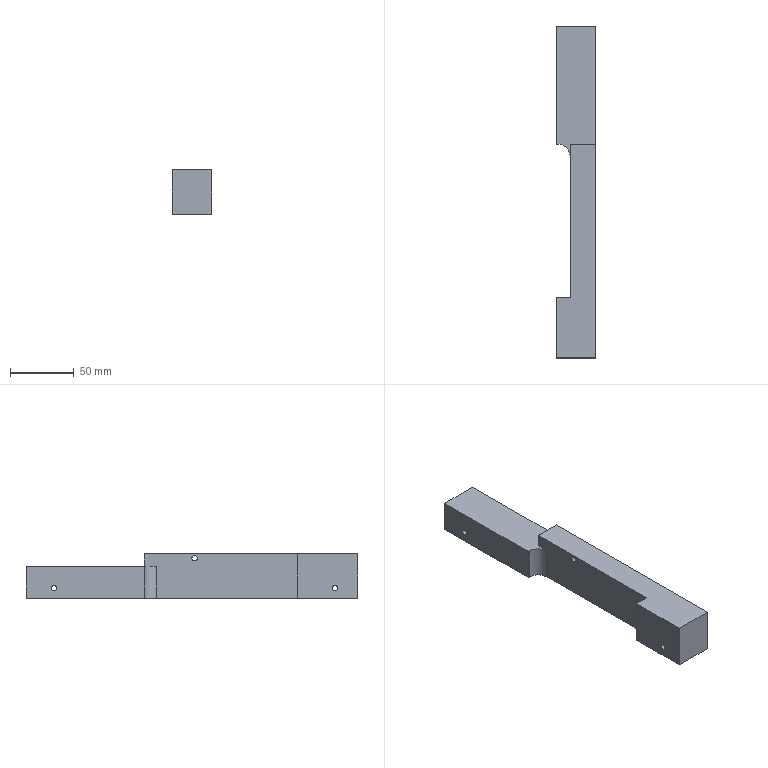Component | SolidWorks | FunnelRotaryCylinderFixingPost-2 | 1 solid | 19 faces | box 31 x 260 x 35 mm | volume 206625 mm3 | plane 12 | cylinder 7 | commonest cylinder face diameters 4.2 x6 20 x1
build123d program:
from build123d import *

# Parameters (mm, degrees)
SKETCH2_W           = 31
SKETCH2_H           = 260
BOSS_EXTRUDE1_DEPTH = 25
SKETCH3_W           = 31
SKETCH3_H           = 167.5
BOSS_EXTRUDE2_DEPTH = 10
M5_TAPPED_HOLE1_D   = 4.2
SKETCH7_W           = 11
SKETCH7_H           = 120
CUT_EXTRUDE1_DEPTH  = 40
FILLET1_R           = 10


with BuildPart() as part:
    # Sketch2 → Boss-Extrude1 (new body)
    with BuildSketch(Plane.XY):
        with Locations((0.5, -69.763)):
            Rectangle(SKETCH2_W, SKETCH2_H)
    extrude(amount=BOSS_EXTRUDE1_DEPTH)

    # Sketch3 → Boss-Extrude2 (add)
    with BuildSketch(Plane(origin=(0, 0, 0), x_dir=(-1, 0, 0), z_dir=(0, 0, -1))):
        with Locations((-0.5, -116.013)):
            Rectangle(SKETCH3_W, SKETCH3_H)
    extrude(amount=BOSS_EXTRUDE2_DEPTH)

    # M5 Tapped Hole1 (through all)
    with Locations(Plane.ZY.offset(15)):
        with Locations((17, 38.237), (-6.5, -71.763), (17, -181.763)):
            Hole(M5_TAPPED_HOLE1_D / 2)

    # Sketch7 → Cut-Extrude1 (cut)
    with BuildSketch(Plane(origin=(0, 0, -10), x_dir=(-1, 0, 0), z_dir=(0, 0, -1))):
        with Locations((-10.5, -92.263)):
            Rectangle(SKETCH7_W, SKETCH7_H)
    extrude(amount=-CUT_EXTRUDE1_DEPTH, mode=Mode.SUBTRACT)

    # Fillet1
    fillet1_edges = [part.edges().sort_by_distance(p)[0] for p in [
        (5, -32.263, 12.5),
    ]]
    fillet(fillet1_edges, radius=FILLET1_R)


solid = part.part

# Placed as in the assembly
solid = solid.moved(Location((-550.496, 52.112, 289.126), (-180, 0, 180)))
STEP:
#1=COLOUR_RGB('',0.7922,0.8196,0.9333);
#2=FILL_AREA_STYLE_COLOUR('',#1);
#3=FILL_AREA_STYLE('',(#2));
#4=SURFACE_STYLE_FILL_AREA(#3);
#5=SURFACE_SIDE_STYLE('',(#4));
#6=SURFACE_STYLE_USAGE(.BOTH.,#5);
#7=PRESENTATION_STYLE_ASSIGNMENT((#6));
#8=CARTESIAN_POINT('',(-22.303,3.557,10.796));
#9=VERTEX_POINT('',#8);
#10=CARTESIAN_POINT('',(-22.303,3.557,10.631));
#11=VERTEX_POINT('',#10);
#12=CARTESIAN_POINT('',(-22.303,3.557,10.714));
#13=DIRECTION('',(1.,0.,0.));
#14=DIRECTION('',(0.,0.,-1.));
#15=AXIS2_PLACEMENT_3D('',#12,#13,#14);
#16=CIRCLE('',#15,0.08268);
#17=EDGE_CURVE('',#9,#11,#16,.T.);
#18=ORIENTED_EDGE('',*,*,#17,.F.);
#19=CARTESIAN_POINT('',(-21.083,3.557,10.796));
#20=VERTEX_POINT('',#19);
#21=CARTESIAN_POINT('',(-21.083,3.557,10.796));
#22=DIRECTION('',(1.,0.,0.));
#23=VECTOR('',#22,39.37);
#24=LINE('',#21,#23);
#25=EDGE_CURVE('',#9,#20,#24,.T.);
#26=ORIENTED_EDGE('',*,*,#25,.T.);
#27=CARTESIAN_POINT('',(-21.083,3.557,10.631));
#28=VERTEX_POINT('',#27);
#29=CARTESIAN_POINT('',(-21.083,3.557,10.714));
#30=DIRECTION('',(1.,0.,0.));
#31=DIRECTION('',(0.,0.,-1.));
#32=AXIS2_PLACEMENT_3D('',#29,#30,#31);
#33=CIRCLE('',#32,0.08268);
#34=EDGE_CURVE('',#20,#28,#33,.T.);
#35=ORIENTED_EDGE('',*,*,#34,.T.);
#36=CARTESIAN_POINT('',(-21.083,3.557,10.631));
#37=DIRECTION('',(1.,0.,0.));
#38=VECTOR('',#37,39.37);
#39=LINE('',#36,#38);
#40=EDGE_CURVE('',#11,#28,#39,.T.);
#41=ORIENTED_EDGE('',*,*,#40,.F.);
#42=EDGE_LOOP('',(#18,#26,#35,#41));
#43=FACE_OUTER_BOUND('',#42,.T.);
#44=CARTESIAN_POINT('',(-21.083,3.557,10.714));
#45=DIRECTION('',(1.,0.,0.));
#46=DIRECTION('',(0.,0.,-1.));
#47=AXIS2_PLACEMENT_3D('',#44,#45,#46);
#48=CYLINDRICAL_SURFACE('',#47,0.08268);
#49=ADVANCED_FACE('',(#43),#48,.F.);
#50=CARTESIAN_POINT('',(-21.87,-0.7737,11.556));
#51=VERTEX_POINT('',#50);
#52=CARTESIAN_POINT('',(-21.87,-0.7737,11.721));
#53=VERTEX_POINT('',#52);
#54=CARTESIAN_POINT('',(-21.87,-0.7737,11.639));
#55=DIRECTION('',(-1.,-0.,-0.));
#56=DIRECTION('',(0.,-1.,0.));
#57=AXIS2_PLACEMENT_3D('',#54,#55,#56);
#58=CIRCLE('',#57,0.08268);
#59=EDGE_CURVE('',#51,#53,#58,.T.);
#60=ORIENTED_EDGE('',*,*,#59,.T.);
#61=CARTESIAN_POINT('',(-21.083,-0.7737,11.721));
#62=VERTEX_POINT('',#61);
#63=CARTESIAN_POINT('',(-21.083,-0.7737,11.721));
#64=DIRECTION('',(1.,0.,0.));
#65=VECTOR('',#64,39.37);
#66=LINE('',#63,#65);
#67=EDGE_CURVE('',#53,#62,#66,.T.);
#68=ORIENTED_EDGE('',*,*,#67,.T.);
#69=CARTESIAN_POINT('',(-21.083,-0.7737,11.556));
#70=VERTEX_POINT('',#69);
#71=CARTESIAN_POINT('',(-21.083,-0.7737,11.639));
#72=DIRECTION('',(1.,0.,0.));
#73=DIRECTION('',(0.,0.,-1.));
#74=AXIS2_PLACEMENT_3D('',#71,#72,#73);
#75=CIRCLE('',#74,0.08268);
#76=EDGE_CURVE('',#62,#70,#75,.T.);
#77=ORIENTED_EDGE('',*,*,#76,.T.);
#78=CARTESIAN_POINT('',(-21.083,-0.7737,11.556));
#79=DIRECTION('',(1.,0.,0.));
#80=VECTOR('',#79,39.37);
#81=LINE('',#78,#80);
#82=EDGE_CURVE('',#51,#70,#81,.T.);
#83=ORIENTED_EDGE('',*,*,#82,.F.);
#84=EDGE_LOOP('',(#60,#68,#77,#83));
#85=FACE_OUTER_BOUND('',#84,.T.);
#86=CARTESIAN_POINT('',(-21.083,-0.7737,11.639));
#87=DIRECTION('',(1.,0.,0.));
#88=DIRECTION('',(0.,0.,-1.));
#89=AXIS2_PLACEMENT_3D('',#86,#87,#88);
#90=CYLINDRICAL_SURFACE('',#89,0.08268);
#91=ADVANCED_FACE('',(#85),#90,.F.);
#92=CARTESIAN_POINT('',(-22.303,-5.104,10.796));
#93=VERTEX_POINT('',#92);
#94=CARTESIAN_POINT('',(-22.303,-5.104,10.631));
#95=VERTEX_POINT('',#94);
#96=CARTESIAN_POINT('',(-22.303,-5.104,10.714));
#97=DIRECTION('',(1.,0.,0.));
#98=DIRECTION('',(0.,0.,-1.));
#99=AXIS2_PLACEMENT_3D('',#96,#97,#98);
#100=CIRCLE('',#99,0.08268);
#101=EDGE_CURVE('',#93,#95,#100,.T.);
#102=ORIENTED_EDGE('',*,*,#101,.F.);
#103=CARTESIAN_POINT('',(-21.083,-5.104,10.796));
#104=VERTEX_POINT('',#103);
#105=CARTESIAN_POINT('',(-21.083,-5.104,10.796));
#106=DIRECTION('',(1.,0.,0.));
#107=VECTOR('',#106,39.37);
#108=LINE('',#105,#107);
#109=EDGE_CURVE('',#93,#104,#108,.T.);
#110=ORIENTED_EDGE('',*,*,#109,.T.);
#111=CARTESIAN_POINT('',(-21.083,-5.104,10.631));
#112=VERTEX_POINT('',#111);
#113=CARTESIAN_POINT('',(-21.083,-5.104,10.714));
#114=DIRECTION('',(1.,0.,0.));
#115=DIRECTION('',(0.,0.,-1.));
#116=AXIS2_PLACEMENT_3D('',#113,#114,#115);
#117=CIRCLE('',#116,0.08268);
#118=EDGE_CURVE('',#104,#112,#117,.T.);
#119=ORIENTED_EDGE('',*,*,#118,.T.);
#120=CARTESIAN_POINT('',(-21.083,-5.104,10.631));
#121=DIRECTION('',(1.,0.,0.));
#122=VECTOR('',#121,39.37);
#123=LINE('',#120,#122);
#124=EDGE_CURVE('',#95,#112,#123,.T.);
#125=ORIENTED_EDGE('',*,*,#124,.F.);
#126=EDGE_LOOP('',(#102,#110,#119,#125));
#127=FACE_OUTER_BOUND('',#126,.T.);
#128=CARTESIAN_POINT('',(-21.083,-5.104,10.714));
#129=DIRECTION('',(1.,0.,0.));
#130=DIRECTION('',(0.,0.,-1.));
#131=AXIS2_PLACEMENT_3D('',#128,#129,#130);
#132=CYLINDRICAL_SURFACE('',#131,0.08268);
#133=ADVANCED_FACE('',(#127),#132,.F.);
#134=CARTESIAN_POINT('',(-22.303,3.557,10.714));
#135=DIRECTION('',(1.,0.,0.));
#136=DIRECTION('',(0.,0.,-1.));
#137=AXIS2_PLACEMENT_3D('',#134,#135,#136);
#138=CIRCLE('',#137,0.08268);
#139=EDGE_CURVE('',#11,#9,#138,.T.);
#140=ORIENTED_EDGE('',*,*,#139,.T.);
#141=ORIENTED_EDGE('',*,*,#17,.T.);
#142=EDGE_LOOP('',(#140,#141));
#143=FACE_BOUND('',#142,.T.);
#144=CARTESIAN_POINT('',(-22.303,0.7814,10.399));
#145=VERTEX_POINT('',#144);
#146=CARTESIAN_POINT('',(-22.303,4.423,10.399));
#147=VERTEX_POINT('',#146);
#148=CARTESIAN_POINT('',(-22.303,4.423,10.399));
#149=DIRECTION('',(0.,1.,-0.));
#150=VECTOR('',#149,39.37);
#151=LINE('',#148,#150);
#152=EDGE_CURVE('',#145,#147,#151,.T.);
#153=ORIENTED_EDGE('',*,*,#152,.F.);
#154=CARTESIAN_POINT('',(-22.303,0.7814,11.383));
#155=VERTEX_POINT('',#154);
#156=CARTESIAN_POINT('',(-22.303,0.7814,10.202));
#157=DIRECTION('',(-0.,0.,1.));
#158=VECTOR('',#157,39.37);
#159=LINE('',#156,#158);
#160=EDGE_CURVE('',#145,#155,#159,.T.);
#161=ORIENTED_EDGE('',*,*,#160,.T.);
#162=CARTESIAN_POINT('',(-22.303,4.423,11.383));
#163=VERTEX_POINT('',#162);
#164=CARTESIAN_POINT('',(-22.303,4.423,11.383));
#165=DIRECTION('',(0.,1.,-0.));
#166=VECTOR('',#165,39.37);
#167=LINE('',#164,#166);
#168=EDGE_CURVE('',#155,#163,#167,.T.);
#169=ORIENTED_EDGE('',*,*,#168,.T.);
#170=CARTESIAN_POINT('',(-22.303,4.423,10.399));
#171=DIRECTION('',(-0.,0.,1.));
#172=VECTOR('',#171,39.37);
#173=LINE('',#170,#172);
#174=EDGE_CURVE('',#147,#163,#173,.T.);
#175=ORIENTED_EDGE('',*,*,#174,.F.);
#176=EDGE_LOOP('',(#153,#161,#169,#175));
#177=FACE_OUTER_BOUND('',#176,.T.);
#178=CARTESIAN_POINT('',(-22.303,4.423,10.399));
#179=DIRECTION('',(1.,-0.,0.));
#180=DIRECTION('',(-0.,-1.,0.));
#181=AXIS2_PLACEMENT_3D('',#178,#179,#180);
#182=PLANE('',#181);
#183=ADVANCED_FACE('',(#143,#177),#182,.F.);
#184=CARTESIAN_POINT('',(-22.303,-5.104,10.714));
#185=DIRECTION('',(1.,0.,0.));
#186=DIRECTION('',(0.,0.,-1.));
#187=AXIS2_PLACEMENT_3D('',#184,#185,#186);
#188=CIRCLE('',#187,0.08268);
#189=EDGE_CURVE('',#95,#93,#188,.T.);
#190=ORIENTED_EDGE('',*,*,#189,.T.);
#191=ORIENTED_EDGE('',*,*,#101,.T.);
#192=EDGE_LOOP('',(#190,#191));
#193=FACE_BOUND('',#192,.T.);
#194=CARTESIAN_POINT('',(-22.303,-3.943,11.777));
#195=VERTEX_POINT('',#194);
#196=CARTESIAN_POINT('',(-22.303,-5.813,11.777));
#197=VERTEX_POINT('',#196);
#198=CARTESIAN_POINT('',(-22.303,-5.813,11.777));
#199=DIRECTION('',(0.,-1.,0.));
#200=VECTOR('',#199,39.37);
#201=LINE('',#198,#200);
#202=EDGE_CURVE('',#195,#197,#201,.T.);
#203=ORIENTED_EDGE('',*,*,#202,.F.);
#204=CARTESIAN_POINT('',(-22.303,-3.943,10.399));
#205=VERTEX_POINT('',#204);
#206=CARTESIAN_POINT('',(-22.303,-3.943,10.202));
#207=DIRECTION('',(-0.,0.,1.));
#208=VECTOR('',#207,39.37);
#209=LINE('',#206,#208);
#210=EDGE_CURVE('',#205,#195,#209,.T.);
#211=ORIENTED_EDGE('',*,*,#210,.F.);
#212=CARTESIAN_POINT('',(-22.303,-5.813,10.399));
#213=VERTEX_POINT('',#212);
#214=CARTESIAN_POINT('',(-22.303,4.423,10.399));
#215=DIRECTION('',(0.,1.,-0.));
#216=VECTOR('',#215,39.37);
#217=LINE('',#214,#216);
#218=EDGE_CURVE('',#213,#205,#217,.T.);
#219=ORIENTED_EDGE('',*,*,#218,.F.);
#220=CARTESIAN_POINT('',(-22.303,-5.813,10.399));
#221=DIRECTION('',(-0.,0.,1.));
#222=VECTOR('',#221,39.37);
#223=LINE('',#220,#222);
#224=EDGE_CURVE('',#213,#197,#223,.T.);
#225=ORIENTED_EDGE('',*,*,#224,.T.);
#226=EDGE_LOOP('',(#203,#211,#219,#225));
#227=FACE_OUTER_BOUND('',#226,.T.);
#228=CARTESIAN_POINT('',(-22.303,4.423,10.399));
#229=DIRECTION('',(1.,-0.,0.));
#230=DIRECTION('',(-0.,-1.,0.));
#231=AXIS2_PLACEMENT_3D('',#228,#229,#230);
#232=PLANE('',#231);
#233=ADVANCED_FACE('',(#193,#227),#232,.F.);
#234=CARTESIAN_POINT('',(-21.083,4.423,11.383));
#235=VERTEX_POINT('',#234);
#236=CARTESIAN_POINT('',(-22.303,4.423,11.383));
#237=DIRECTION('',(1.,-0.,0.));
#238=VECTOR('',#237,39.37);
#239=LINE('',#236,#238);
#240=EDGE_CURVE('',#163,#235,#239,.T.);
#241=ORIENTED_EDGE('',*,*,#240,.T.);
#242=CARTESIAN_POINT('',(-21.083,4.423,10.399));
#243=VERTEX_POINT('',#242);
#244=CARTESIAN_POINT('',(-21.083,4.423,10.399));
#245=DIRECTION('',(-0.,0.,1.));
#246=VECTOR('',#245,39.37);
#247=LINE('',#244,#246);
#248=EDGE_CURVE('',#243,#235,#247,.T.);
#249=ORIENTED_EDGE('',*,*,#248,.F.);
#250=CARTESIAN_POINT('',(-22.303,4.423,10.399));
#251=DIRECTION('',(1.,-0.,0.));
#252=VECTOR('',#251,39.37);
#253=LINE('',#250,#252);
#254=EDGE_CURVE('',#147,#243,#253,.T.);
#255=ORIENTED_EDGE('',*,*,#254,.F.);
#256=ORIENTED_EDGE('',*,*,#174,.T.);
#257=EDGE_LOOP('',(#241,#249,#255,#256));
#258=FACE_OUTER_BOUND('',#257,.T.);
#259=CARTESIAN_POINT('',(-22.303,4.423,10.399));
#260=DIRECTION('',(-0.,-1.,0.));
#261=DIRECTION('',(-1.,0.,-0.));
#262=AXIS2_PLACEMENT_3D('',#259,#260,#261);
#263=PLANE('',#262);
#264=ADVANCED_FACE('',(#258),#263,.F.);
#265=CARTESIAN_POINT('',(-21.083,3.557,10.714));
#266=DIRECTION('',(1.,0.,0.));
#267=DIRECTION('',(0.,0.,-1.));
#268=AXIS2_PLACEMENT_3D('',#265,#266,#267);
#269=CIRCLE('',#268,0.08268);
#270=EDGE_CURVE('',#28,#20,#269,.T.);
#271=ORIENTED_EDGE('',*,*,#270,.F.);
#272=ORIENTED_EDGE('',*,*,#34,.F.);
#273=EDGE_LOOP('',(#271,#272));
#274=FACE_BOUND('',#273,.T.);
#275=CARTESIAN_POINT('',(-21.083,-0.7737,11.639));
#276=DIRECTION('',(1.,0.,0.));
#277=DIRECTION('',(0.,0.,-1.));
#278=AXIS2_PLACEMENT_3D('',#275,#276,#277);
#279=CIRCLE('',#278,0.08268);
#280=EDGE_CURVE('',#70,#62,#279,.T.);
#281=ORIENTED_EDGE('',*,*,#280,.F.);
#282=ORIENTED_EDGE('',*,*,#76,.F.);
#283=EDGE_LOOP('',(#281,#282));
#284=FACE_BOUND('',#283,.T.);
#285=CARTESIAN_POINT('',(-21.083,-5.104,10.714));
#286=DIRECTION('',(1.,0.,0.));
#287=DIRECTION('',(0.,0.,-1.));
#288=AXIS2_PLACEMENT_3D('',#285,#286,#287);
#289=CIRCLE('',#288,0.08268);
#290=EDGE_CURVE('',#112,#104,#289,.T.);
#291=ORIENTED_EDGE('',*,*,#290,.F.);
#292=ORIENTED_EDGE('',*,*,#118,.F.);
#293=EDGE_LOOP('',(#291,#292));
#294=FACE_BOUND('',#293,.T.);
#295=CARTESIAN_POINT('',(-21.083,0.7814,11.383));
#296=VERTEX_POINT('',#295);
#297=CARTESIAN_POINT('',(-21.083,4.423,11.383));
#298=DIRECTION('',(-0.,-1.,0.));
#299=VECTOR('',#298,39.37);
#300=LINE('',#297,#299);
#301=EDGE_CURVE('',#235,#296,#300,.T.);
#302=ORIENTED_EDGE('',*,*,#301,.T.);
#303=CARTESIAN_POINT('',(-21.083,0.7814,11.777));
#304=VERTEX_POINT('',#303);
#305=CARTESIAN_POINT('',(-21.083,0.7814,11.777));
#306=DIRECTION('',(0.,-0.,-1.));
#307=VECTOR('',#306,39.37);
#308=LINE('',#305,#307);
#309=EDGE_CURVE('',#304,#296,#308,.T.);
#310=ORIENTED_EDGE('',*,*,#309,.F.);
#311=CARTESIAN_POINT('',(-21.083,-5.813,11.777));
#312=VERTEX_POINT('',#311);
#313=CARTESIAN_POINT('',(-21.083,-5.813,11.777));
#314=DIRECTION('',(0.,1.,-0.));
#315=VECTOR('',#314,39.37);
#316=LINE('',#313,#315);
#317=EDGE_CURVE('',#312,#304,#316,.T.);
#318=ORIENTED_EDGE('',*,*,#317,.F.);
#319=CARTESIAN_POINT('',(-21.083,-5.813,10.399));
#320=VERTEX_POINT('',#319);
#321=CARTESIAN_POINT('',(-21.083,-5.813,10.399));
#322=DIRECTION('',(-0.,0.,1.));
#323=VECTOR('',#322,39.37);
#324=LINE('',#321,#323);
#325=EDGE_CURVE('',#320,#312,#324,.T.);
#326=ORIENTED_EDGE('',*,*,#325,.F.);
#327=CARTESIAN_POINT('',(-21.083,4.423,10.399));
#328=DIRECTION('',(-0.,-1.,0.));
#329=VECTOR('',#328,39.37);
#330=LINE('',#327,#329);
#331=EDGE_CURVE('',#243,#320,#330,.T.);
#332=ORIENTED_EDGE('',*,*,#331,.F.);
#333=ORIENTED_EDGE('',*,*,#248,.T.);
#334=EDGE_LOOP('',(#302,#310,#318,#326,#332,#333));
#335=FACE_OUTER_BOUND('',#334,.T.);
#336=CARTESIAN_POINT('',(-21.083,4.423,10.399));
#337=DIRECTION('',(-1.,0.,-0.));
#338=DIRECTION('',(0.,1.,-0.));
#339=AXIS2_PLACEMENT_3D('',#336,#337,#338);
#340=PLANE('',#339);
#341=ADVANCED_FACE('',(#274,#284,#294,#335),#340,.F.);
#342=ORIENTED_EDGE('',*,*,#325,.T.);
#343=CARTESIAN_POINT('',(-22.303,-5.813,11.777));
#344=DIRECTION('',(1.,0.,0.));
#345=VECTOR('',#344,39.37);
#346=LINE('',#343,#345);
#347=EDGE_CURVE('',#197,#312,#346,.T.);
#348=ORIENTED_EDGE('',*,*,#347,.F.);
#349=ORIENTED_EDGE('',*,*,#224,.F.);
#350=CARTESIAN_POINT('',(-22.303,-5.813,10.399));
#351=DIRECTION('',(-1.,-0.,-0.));
#352=VECTOR('',#351,39.37);
#353=LINE('',#350,#352);
#354=EDGE_CURVE('',#320,#213,#353,.T.);
#355=ORIENTED_EDGE('',*,*,#354,.F.);
#356=EDGE_LOOP('',(#342,#348,#349,#355));
#357=FACE_OUTER_BOUND('',#356,.T.);
#358=CARTESIAN_POINT('',(-22.303,-5.813,10.399));
#359=DIRECTION('',(0.,1.,-0.));
#360=DIRECTION('',(0.,-0.,-1.));
#361=AXIS2_PLACEMENT_3D('',#358,#359,#360);
#362=PLANE('',#361);
#363=ADVANCED_FACE('',(#357),#362,.F.);
#364=CARTESIAN_POINT('',(-21.87,-3.943,10.399));
#365=VERTEX_POINT('',#364);
#366=CARTESIAN_POINT('',(-21.87,0.3877,10.399));
#367=VERTEX_POINT('',#366);
#368=CARTESIAN_POINT('',(-21.87,2.052,10.399));
#369=DIRECTION('',(-0.,1.,-0.));
#370=VECTOR('',#369,39.37);
#371=LINE('',#368,#370);
#372=EDGE_CURVE('',#365,#367,#371,.T.);
#373=ORIENTED_EDGE('',*,*,#372,.T.);
#374=CARTESIAN_POINT('',(-22.264,0.7814,10.399));
#375=VERTEX_POINT('',#374);
#376=CARTESIAN_POINT('',(-22.264,0.3877,10.399));
#377=DIRECTION('',(-0.,0.,1.));
#378=DIRECTION('',(1.,0.,0.));
#379=AXIS2_PLACEMENT_3D('',#376,#377,#378);
#380=CIRCLE('',#379,0.3937);
#381=EDGE_CURVE('',#367,#375,#380,.T.);
#382=ORIENTED_EDGE('',*,*,#381,.T.);
#383=CARTESIAN_POINT('',(-21.673,0.7814,10.399));
#384=DIRECTION('',(-1.,-0.,-0.));
#385=VECTOR('',#384,39.37);
#386=LINE('',#383,#385);
#387=EDGE_CURVE('',#375,#145,#386,.T.);
#388=ORIENTED_EDGE('',*,*,#387,.T.);
#389=ORIENTED_EDGE('',*,*,#152,.T.);
#390=ORIENTED_EDGE('',*,*,#254,.T.);
#391=ORIENTED_EDGE('',*,*,#331,.T.);
#392=ORIENTED_EDGE('',*,*,#354,.T.);
#393=ORIENTED_EDGE('',*,*,#218,.T.);
#394=CARTESIAN_POINT('',(-21.673,-3.943,10.399));
#395=DIRECTION('',(1.,0.,0.));
#396=VECTOR('',#395,39.37);
#397=LINE('',#394,#396);
#398=EDGE_CURVE('',#205,#365,#397,.T.);
#399=ORIENTED_EDGE('',*,*,#398,.T.);
#400=EDGE_LOOP('',(#373,#382,#388,#389,#390,#391,#392,#393,#399));
#401=FACE_OUTER_BOUND('',#400,.T.);
#402=CARTESIAN_POINT('',(-21.673,2.052,10.399));
#403=DIRECTION('',(-0.,0.,1.));
#404=DIRECTION('',(1.,0.,0.));
#405=AXIS2_PLACEMENT_3D('',#402,#403,#404);
#406=PLANE('',#405);
#407=ADVANCED_FACE('',(#401),#406,.F.);
#408=CARTESIAN_POINT('',(-21.87,0.7814,11.383));
#409=VERTEX_POINT('',#408);
#410=CARTESIAN_POINT('',(-22.303,0.7814,11.383));
#411=DIRECTION('',(-1.,-0.,-0.));
#412=VECTOR('',#411,39.37);
#413=LINE('',#410,#412);
#414=EDGE_CURVE('',#296,#409,#413,.T.);
#415=ORIENTED_EDGE('',*,*,#414,.F.);
#416=ORIENTED_EDGE('',*,*,#301,.F.);
#417=ORIENTED_EDGE('',*,*,#240,.F.);
#418=ORIENTED_EDGE('',*,*,#168,.F.);
#419=CARTESIAN_POINT('',(-22.264,0.7814,11.383));
#420=VERTEX_POINT('',#419);
#421=CARTESIAN_POINT('',(-21.673,0.7814,11.383));
#422=DIRECTION('',(-1.,-0.,-0.));
#423=VECTOR('',#422,39.37);
#424=LINE('',#421,#423);
#425=EDGE_CURVE('',#420,#155,#424,.T.);
#426=ORIENTED_EDGE('',*,*,#425,.F.);
#427=CARTESIAN_POINT('',(-21.87,0.3877,11.383));
#428=VERTEX_POINT('',#427);
#429=CARTESIAN_POINT('',(-22.264,0.3877,11.383));
#430=DIRECTION('',(0.,-0.,-1.));
#431=DIRECTION('',(1.,0.,0.));
#432=AXIS2_PLACEMENT_3D('',#429,#430,#431);
#433=CIRCLE('',#432,0.3937);
#434=EDGE_CURVE('',#420,#428,#433,.T.);
#435=ORIENTED_EDGE('',*,*,#434,.T.);
#436=CARTESIAN_POINT('',(-21.87,0.7814,11.383));
#437=DIRECTION('',(0.,-1.,0.));
#438=VECTOR('',#437,39.37);
#439=LINE('',#436,#438);
#440=EDGE_CURVE('',#409,#428,#439,.T.);
#441=ORIENTED_EDGE('',*,*,#440,.F.);
#442=EDGE_LOOP('',(#415,#416,#417,#418,#426,#435,#441));
#443=FACE_OUTER_BOUND('',#442,.T.);
#444=CARTESIAN_POINT('',(-21.673,2.052,11.383));
#445=DIRECTION('',(-0.,0.,1.));
#446=DIRECTION('',(1.,0.,0.));
#447=AXIS2_PLACEMENT_3D('',#444,#445,#446);
#448=PLANE('',#447);
#449=ADVANCED_FACE('',(#443),#448,.T.);
#450=ORIENTED_EDGE('',*,*,#414,.T.);
#451=CARTESIAN_POINT('',(-21.87,0.7814,11.777));
#452=VERTEX_POINT('',#451);
#453=CARTESIAN_POINT('',(-21.87,0.7814,10.202));
#454=DIRECTION('',(-0.,0.,1.));
#455=VECTOR('',#454,39.37);
#456=LINE('',#453,#455);
#457=EDGE_CURVE('',#409,#452,#456,.T.);
#458=ORIENTED_EDGE('',*,*,#457,.T.);
#459=CARTESIAN_POINT('',(-22.303,0.7814,11.777));
#460=DIRECTION('',(-1.,-0.,-0.));
#461=VECTOR('',#460,39.37);
#462=LINE('',#459,#461);
#463=EDGE_CURVE('',#304,#452,#462,.T.);
#464=ORIENTED_EDGE('',*,*,#463,.F.);
#465=ORIENTED_EDGE('',*,*,#309,.T.);
#466=EDGE_LOOP('',(#450,#458,#464,#465));
#467=FACE_OUTER_BOUND('',#466,.T.);
#468=CARTESIAN_POINT('',(-22.303,0.7814,11.777));
#469=DIRECTION('',(0.,-1.,0.));
#470=DIRECTION('',(-0.,0.,1.));
#471=AXIS2_PLACEMENT_3D('',#468,#469,#470);
#472=PLANE('',#471);
#473=ADVANCED_FACE('',(#467),#472,.F.);
#474=ORIENTED_EDGE('',*,*,#463,.T.);
#475=CARTESIAN_POINT('',(-21.87,-3.943,11.777));
#476=VERTEX_POINT('',#475);
#477=CARTESIAN_POINT('',(-21.87,0.7814,11.777));
#478=DIRECTION('',(-0.,1.,-0.));
#479=VECTOR('',#478,39.37);
#480=LINE('',#477,#479);
#481=EDGE_CURVE('',#476,#452,#480,.T.);
#482=ORIENTED_EDGE('',*,*,#481,.F.);
#483=CARTESIAN_POINT('',(-22.303,-3.943,11.777));
#484=DIRECTION('',(1.,0.,0.));
#485=VECTOR('',#484,39.37);
#486=LINE('',#483,#485);
#487=EDGE_CURVE('',#195,#476,#486,.T.);
#488=ORIENTED_EDGE('',*,*,#487,.F.);
#489=ORIENTED_EDGE('',*,*,#202,.T.);
#490=ORIENTED_EDGE('',*,*,#347,.T.);
#491=ORIENTED_EDGE('',*,*,#317,.T.);
#492=EDGE_LOOP('',(#474,#482,#488,#489,#490,#491));
#493=FACE_OUTER_BOUND('',#492,.T.);
#494=CARTESIAN_POINT('',(-21.673,2.052,11.777));
#495=DIRECTION('',(0.,-0.,-1.));
#496=DIRECTION('',(-1.,-0.,-0.));
#497=AXIS2_PLACEMENT_3D('',#494,#495,#496);
#498=PLANE('',#497);
#499=ADVANCED_FACE('',(#493),#498,.F.);
#500=ORIENTED_EDGE('',*,*,#109,.F.);
#501=ORIENTED_EDGE('',*,*,#189,.F.);
#502=ORIENTED_EDGE('',*,*,#124,.T.);
#503=ORIENTED_EDGE('',*,*,#290,.T.);
#504=EDGE_LOOP('',(#500,#501,#502,#503));
#505=FACE_OUTER_BOUND('',#504,.T.);
#506=CARTESIAN_POINT('',(-21.083,-5.104,10.714));
#507=DIRECTION('',(1.,0.,0.));
#508=DIRECTION('',(0.,0.,-1.));
#509=AXIS2_PLACEMENT_3D('',#506,#507,#508);
#510=CYLINDRICAL_SURFACE('',#509,0.08268);
#511=ADVANCED_FACE('',(#505),#510,.F.);
#512=ORIENTED_EDGE('',*,*,#67,.F.);
#513=CARTESIAN_POINT('',(-21.87,-0.7737,11.639));
#514=DIRECTION('',(-1.,-0.,-0.));
#515=DIRECTION('',(0.,-1.,0.));
#516=AXIS2_PLACEMENT_3D('',#513,#514,#515);
#517=CIRCLE('',#516,0.08268);
#518=EDGE_CURVE('',#53,#51,#517,.T.);
#519=ORIENTED_EDGE('',*,*,#518,.T.);
#520=ORIENTED_EDGE('',*,*,#82,.T.);
#521=ORIENTED_EDGE('',*,*,#280,.T.);
#522=EDGE_LOOP('',(#512,#519,#520,#521));
#523=FACE_OUTER_BOUND('',#522,.T.);
#524=CARTESIAN_POINT('',(-21.083,-0.7737,11.639));
#525=DIRECTION('',(1.,0.,0.));
#526=DIRECTION('',(0.,0.,-1.));
#527=AXIS2_PLACEMENT_3D('',#524,#525,#526);
#528=CYLINDRICAL_SURFACE('',#527,0.08268);
#529=ADVANCED_FACE('',(#523),#528,.F.);
#530=ORIENTED_EDGE('',*,*,#25,.F.);
#531=ORIENTED_EDGE('',*,*,#139,.F.);
#532=ORIENTED_EDGE('',*,*,#40,.T.);
#533=ORIENTED_EDGE('',*,*,#270,.T.);
#534=EDGE_LOOP('',(#530,#531,#532,#533));
#535=FACE_OUTER_BOUND('',#534,.T.);
#536=CARTESIAN_POINT('',(-21.083,3.557,10.714));
#537=DIRECTION('',(1.,0.,0.));
#538=DIRECTION('',(0.,0.,-1.));
#539=AXIS2_PLACEMENT_3D('',#536,#537,#538);
#540=CYLINDRICAL_SURFACE('',#539,0.08268);
#541=ADVANCED_FACE('',(#535),#540,.F.);
#542=ORIENTED_EDGE('',*,*,#387,.F.);
#543=CARTESIAN_POINT('',(-22.264,0.7814,11.383));
#544=DIRECTION('',(-0.,0.,1.));
#545=VECTOR('',#544,39.37);
#546=LINE('',#543,#545);
#547=EDGE_CURVE('',#375,#420,#546,.T.);
#548=ORIENTED_EDGE('',*,*,#547,.T.);
#549=ORIENTED_EDGE('',*,*,#425,.T.);
#550=ORIENTED_EDGE('',*,*,#160,.F.);
#551=EDGE_LOOP('',(#542,#548,#549,#550));
#552=FACE_OUTER_BOUND('',#551,.T.);
#553=CARTESIAN_POINT('',(-22.303,0.7814,10.202));
#554=DIRECTION('',(0.,1.,-0.));
#555=DIRECTION('',(0.,-0.,-1.));
#556=AXIS2_PLACEMENT_3D('',#553,#554,#555);
#557=PLANE('',#556);
#558=ADVANCED_FACE('',(#552),#557,.F.);
#559=ORIENTED_EDGE('',*,*,#210,.T.);
#560=ORIENTED_EDGE('',*,*,#487,.T.);
#561=CARTESIAN_POINT('',(-21.87,-3.943,10.202));
#562=DIRECTION('',(-0.,0.,1.));
#563=VECTOR('',#562,39.37);
#564=LINE('',#561,#563);
#565=EDGE_CURVE('',#365,#476,#564,.T.);
#566=ORIENTED_EDGE('',*,*,#565,.F.);
#567=ORIENTED_EDGE('',*,*,#398,.F.);
#568=EDGE_LOOP('',(#559,#560,#566,#567));
#569=FACE_OUTER_BOUND('',#568,.T.);
#570=CARTESIAN_POINT('',(-22.303,-3.943,10.202));
#571=DIRECTION('',(0.,-1.,0.));
#572=DIRECTION('',(-0.,0.,1.));
#573=AXIS2_PLACEMENT_3D('',#570,#571,#572);
#574=PLANE('',#573);
#575=ADVANCED_FACE('',(#569),#574,.F.);
#576=ORIENTED_EDGE('',*,*,#59,.F.);
#577=ORIENTED_EDGE('',*,*,#518,.F.);
#578=EDGE_LOOP('',(#576,#577));
#579=FACE_BOUND('',#578,.T.);
#580=ORIENTED_EDGE('',*,*,#457,.F.);
#581=ORIENTED_EDGE('',*,*,#440,.T.);
#582=CARTESIAN_POINT('',(-21.87,0.3877,10.399));
#583=DIRECTION('',(0.,-0.,-1.));
#584=VECTOR('',#583,39.37);
#585=LINE('',#582,#584);
#586=EDGE_CURVE('',#428,#367,#585,.T.);
#587=ORIENTED_EDGE('',*,*,#586,.T.);
#588=ORIENTED_EDGE('',*,*,#372,.F.);
#589=ORIENTED_EDGE('',*,*,#565,.T.);
#590=ORIENTED_EDGE('',*,*,#481,.T.);
#591=EDGE_LOOP('',(#580,#581,#587,#588,#589,#590));
#592=FACE_OUTER_BOUND('',#591,.T.);
#593=CARTESIAN_POINT('',(-21.87,0.7814,10.202));
#594=DIRECTION('',(1.,0.,0.));
#595=DIRECTION('',(0.,-1.,0.));
#596=AXIS2_PLACEMENT_3D('',#593,#594,#595);
#597=PLANE('',#596);
#598=ADVANCED_FACE('',(#579,#592),#597,.F.);
#599=ORIENTED_EDGE('',*,*,#381,.F.);
#600=ORIENTED_EDGE('',*,*,#586,.F.);
#601=ORIENTED_EDGE('',*,*,#434,.F.);
#602=ORIENTED_EDGE('',*,*,#547,.F.);
#603=EDGE_LOOP('',(#599,#600,#601,#602));
#604=FACE_OUTER_BOUND('',#603,.T.);
#605=CARTESIAN_POINT('',(-22.264,0.3877,10.202));
#606=DIRECTION('',(0.,-0.,-1.));
#607=DIRECTION('',(-1.,0.,0.));
#608=AXIS2_PLACEMENT_3D('',#605,#606,#607);
#609=CYLINDRICAL_SURFACE('',#608,0.3937);
#610=ADVANCED_FACE('',(#604),#609,.F.);
#611=CLOSED_SHELL('',(#49,#91,#133,#183,#233,#264,#341,#363,#407,#449,#473,#499,#511,#529,#541,#558,#575,#598,#610));
#612=MANIFOLD_SOLID_BREP('',#611);
#613=STYLED_ITEM('',(#7),#612);
#614=PRESENTATION_LAYER_ASSIGNMENT('','',(#613));
#615=CARTESIAN_POINT('',(0.,0.,0.));
#616=DIRECTION('',(0.,0.,1.));
#617=DIRECTION('',(1.,0.,0.));
#618=AXIS2_PLACEMENT_3D('',#615,#616,#617);
#619=(LENGTH_UNIT()NAMED_UNIT(*)SI_UNIT($,.METRE.));
#620=LENGTH_MEASURE_WITH_UNIT(LENGTH_MEASURE(0.0254),#619);
#621=DIMENSIONAL_EXPONENTS(1.,0.,0.,0.,0.,0.,0.);
#622=(CONVERSION_BASED_UNIT('',#620)LENGTH_UNIT()NAMED_UNIT(#621));
#623=UNCERTAINTY_MEASURE_WITH_UNIT(LENGTH_MEASURE(0.00001),#622,'','');
#624=(NAMED_UNIT(*)PLANE_ANGLE_UNIT()SI_UNIT($,.RADIAN.));
#625=(NAMED_UNIT(*)SI_UNIT($,.STERADIAN.)SOLID_ANGLE_UNIT());
#626=(GEOMETRIC_REPRESENTATION_CONTEXT(3)GLOBAL_UNCERTAINTY_ASSIGNED_CONTEXT((#623))GLOBAL_UNIT_ASSIGNED_CONTEXT((#622,#624,#625))REPRESENTATION_CONTEXT('',''));
#627=ADVANCED_BREP_SHAPE_REPRESENTATION('',(#612,#618),#626);
#628=(LENGTH_UNIT()NAMED_UNIT(*)SI_UNIT($,.METRE.));
#629=LENGTH_MEASURE_WITH_UNIT(LENGTH_MEASURE(0.0254),#628);
#630=DIMENSIONAL_EXPONENTS(1.,0.,0.,0.,0.,0.,0.);
#631=(CONVERSION_BASED_UNIT('',#629)LENGTH_UNIT()NAMED_UNIT(#630));
#632=UNCERTAINTY_MEASURE_WITH_UNIT(LENGTH_MEASURE(0.00001),#631,'','');
#633=(NAMED_UNIT(*)PLANE_ANGLE_UNIT()SI_UNIT($,.RADIAN.));
#634=(NAMED_UNIT(*)SI_UNIT($,.STERADIAN.)SOLID_ANGLE_UNIT());
#635=(GEOMETRIC_REPRESENTATION_CONTEXT(3)GLOBAL_UNCERTAINTY_ASSIGNED_CONTEXT((#632))GLOBAL_UNIT_ASSIGNED_CONTEXT((#631,#633,#634))REPRESENTATION_CONTEXT('',''));
#636=MECHANICAL_DESIGN_GEOMETRIC_PRESENTATION_REPRESENTATION('',(#613),#635);